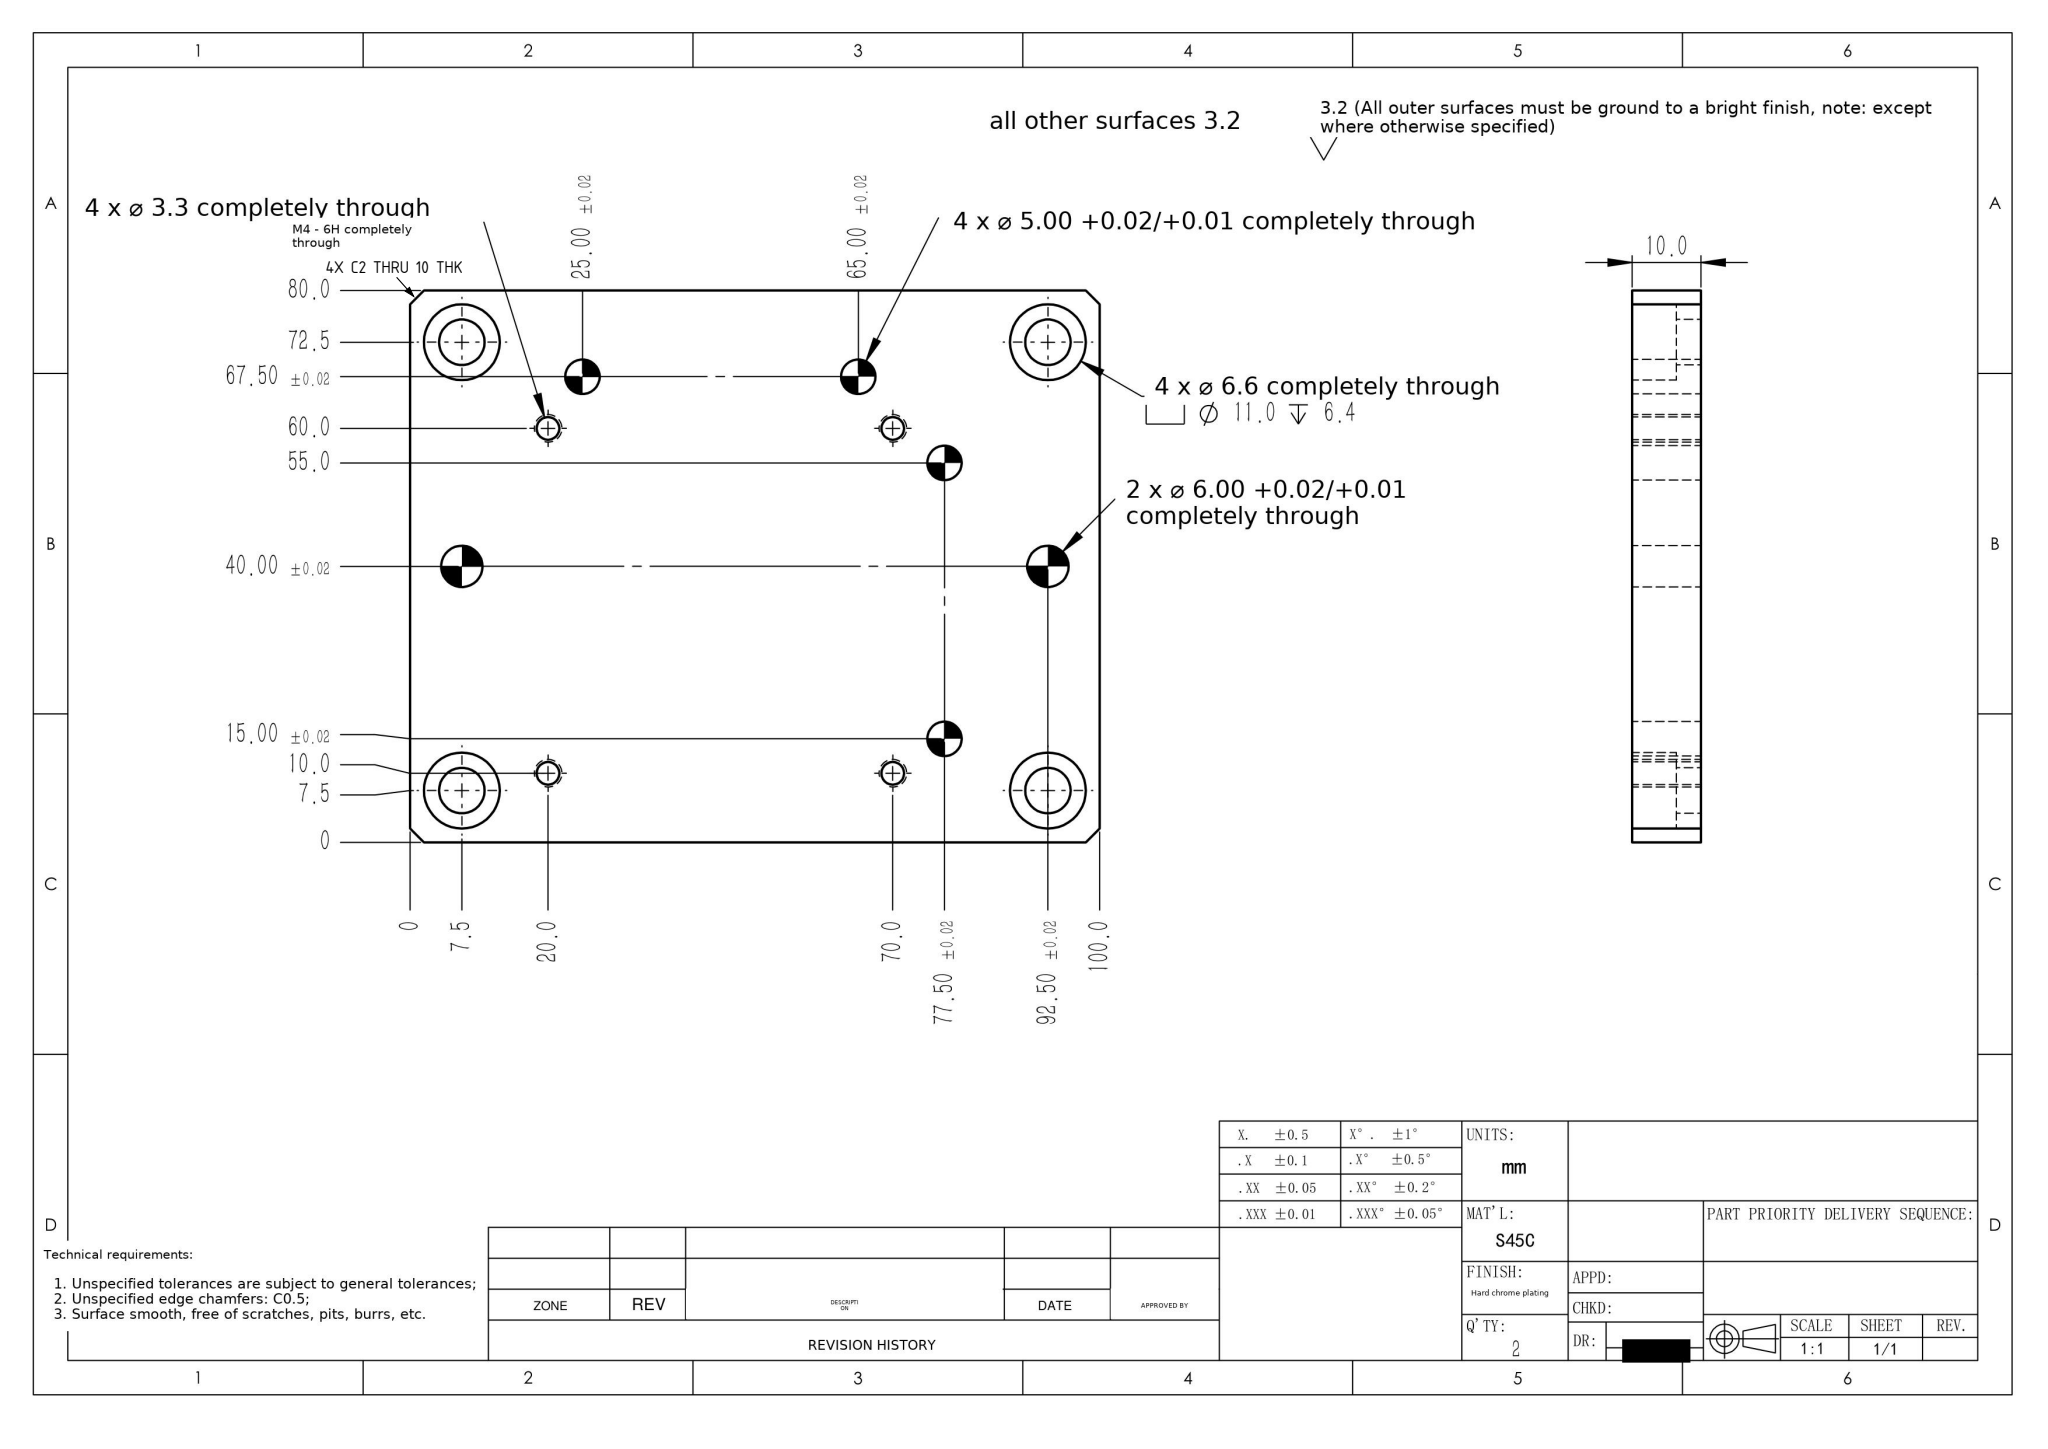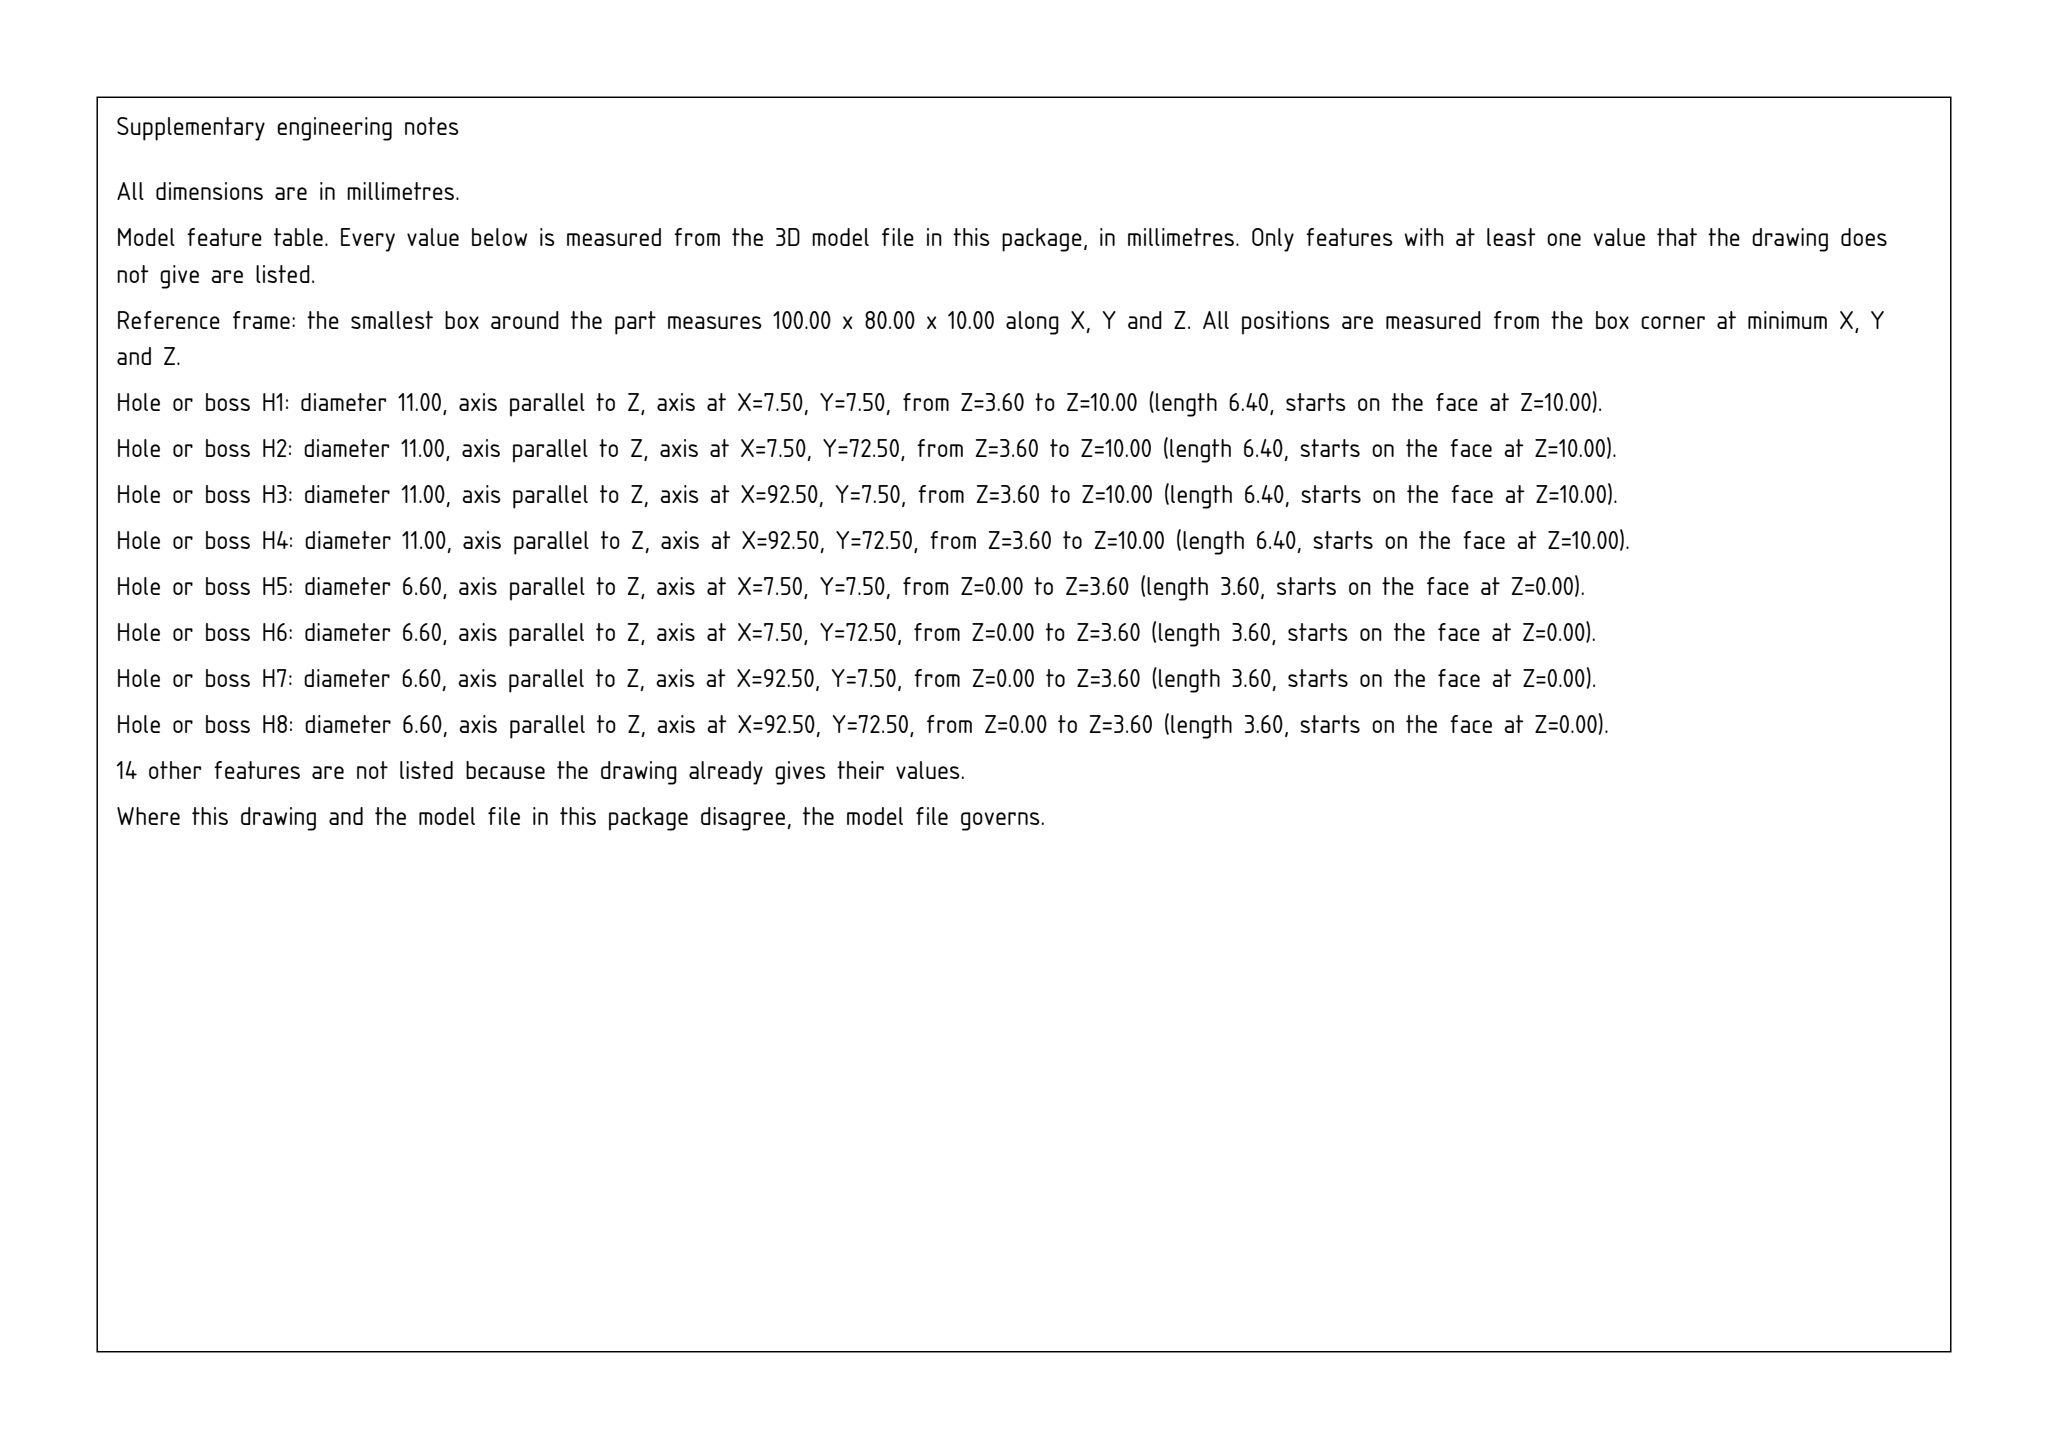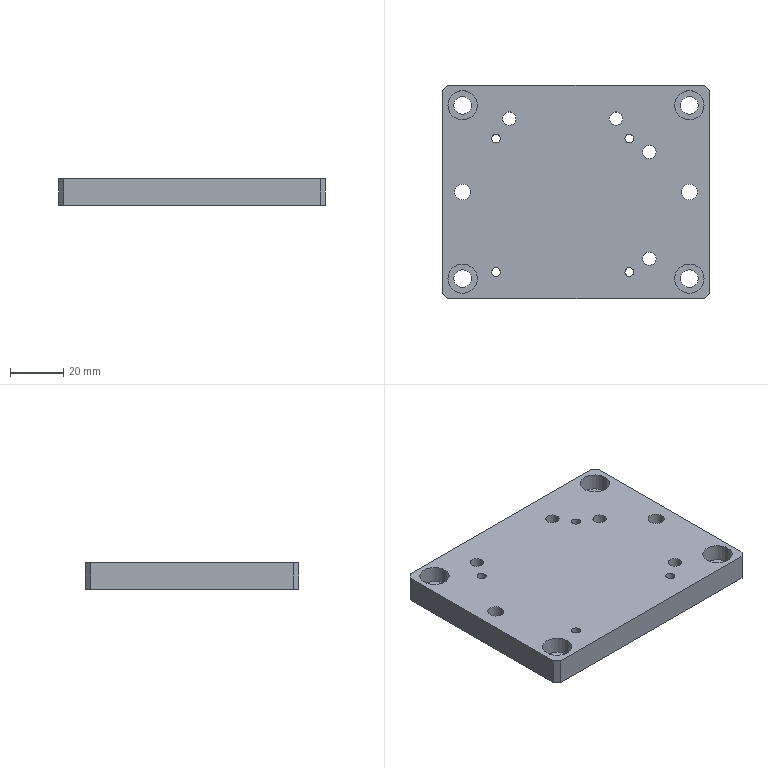Part | SolidWorks | mm | material S45C | 1 solid | 50 faces | box 100 x 80 x 10 mm | volume 75301 mm3 | cylinder 36 | plane 14 | commonest cylinder face diameters 5 x8 11 x8 6.6 x8 3.3 x8 6 x4
Drawing notes:
4X CORNER CHAMFER C2 (2.0 x 45°) THRU 10 THK | from the solid: 4 inclined planes at 45° to X and Y, size 2.0 x 2.0 x 10.0, at bbox corners [0,0],[0,78],[98,0],[98,78]; plate 100x80x10
build123d program:
from build123d import *

# Parameters (mm, degrees)
SKETCH1_W                                       = 100
SKETCH1_H                                       = 80
BOSS_EXTRUDE1_DEPTH                             = 10
M4_TAPPED_HOLE1_D                               = 3.3
M6_HEX_SOCKET_HEAD_CAP_SCREW_CBORE1_D           = 6.6
M6_HEX_SOCKET_HEAD_CAP_SCREW_CBORE1_CBORE_D     = 11
M6_HEX_SOCKET_HEAD_CAP_SCREW_CBORE1_CBORE_DEPTH = 6.4
SIZE_MM_DOWEL_PIN_HOLE1_D                       = 6
SIZE_MM_DOWEL_PIN_HOLE2_D                       = 5
CHAMFER1_SIZE                                   = 2


with BuildPart() as part:
    # Sketch1 → Boss-Extrude1 (new body)
    with BuildSketch(Plane.XY):
        Rectangle(SKETCH1_W, SKETCH1_H)
    extrude(amount=BOSS_EXTRUDE1_DEPTH)

    # M4 Tapped Hole1 (through all)
    with Locations(Plane.XY.offset(10)):
        with Locations((-30, -30), (20, -30), (20, 20), (-30, 20)):
            Hole(M4_TAPPED_HOLE1_D / 2)

    # M6 Hex Socket Head Cap Screw CBORE1 (through all)
    with Locations(Plane.XY.offset(10)):
        with Locations((-42.5, -32.5), (42.5, -32.5), (42.5, 32.5), (-42.5, 32.5)):
            CounterBoreHole(M6_HEX_SOCKET_HEAD_CAP_SCREW_CBORE1_D / 2, M6_HEX_SOCKET_HEAD_CAP_SCREW_CBORE1_CBORE_D / 2, M6_HEX_SOCKET_HEAD_CAP_SCREW_CBORE1_CBORE_DEPTH)

    # Size mm Dowel Pin Hole1 (through all)
    with Locations(Plane.XY.offset(10)):
        with Locations((-42.5, 0), (42.5, 0)):
            Hole(SIZE_MM_DOWEL_PIN_HOLE1_D / 2)

    # Size mm Dowel Pin Hole2 (through all)
    with Locations(Plane.XY.offset(10)):
        with Locations((-25, 27.5), (15, 27.5), (27.5, 15), (27.5, -25)):
            Hole(SIZE_MM_DOWEL_PIN_HOLE2_D / 2)

    # Chamfer1
    chamfer1_edges = [part.edges().sort_by_distance(p)[0] for p in [
        (50, -40, 5),
        (-50, -40, 5),
        (-50, 40, 5),
        (50, 40, 5),
    ]]
    chamfer(chamfer1_edges, length=CHAMFER1_SIZE)


solid = part.part